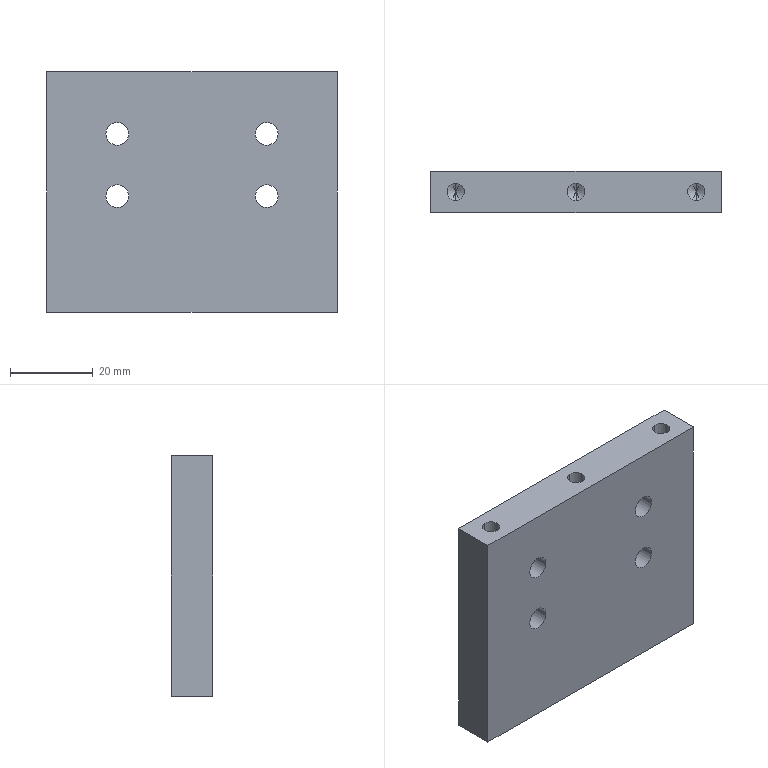Component | SolidWorks | LD101-02--Q1000-Q16-1.SLDQ1SM-1_LD101-02--Q1109-1-2 | 1 solid | 50 faces | box 70 x 10 x 58 mm | volume 37509 mm3 | cylinder 28 | cone 12 | plane 10 | commonest cylinder face diameters 4.2 x12 9 x8 5.5 x8 | material AL6061
build123d program:
from build123d import *

# Parameters (mm, degrees)
SKETCH1_W                                          = 70
SKETCH1_H                                          = 58
BOSS_EXTRUDE1_DEPTH                                = 5
M5_TAPPED_HOLE1_AT_2_COUNT                         = 2
M5_TAPPED_HOLE1_AT_2_PITCH                         = 58
M5_TAPPED_HOLE1_AT_3_COUNT                         = 2
M5_TAPPED_HOLE1_AT_3_PITCH                         = 29
HOLE_SIZE_FOR_HEX_SOCKET_HEAD_CAP_SCRE_D           = 5.5
HOLE_SIZE_FOR_HEX_SOCKET_HEAD_CAP_SCRE_CBORE_D     = 9
HOLE_SIZE_FOR_HEX_SOCKET_HEAD_CAP_SCRE_CBORE_DEPTH = 5.7


with BuildPart() as part:
    # Sketch1 → Boss-Extrude1 (new, symmetric)
    with BuildSketch(Plane.XY):
        Rectangle(SKETCH1_W, SKETCH1_H)
    extrude(amount=BOSS_EXTRUDE1_DEPTH, both=True)

    # Sketch2 → M5 Tapped Hole1 (revolve, cut)
    with BuildSketch(Plane(origin=(-29, 29, 0), x_dir=(0, 0, 1), z_dir=(1, 0, 0))):
        Polygon((0, 0), (0, 15.662), (2.1, 14.4), (2.1, 0), align=None)
    m5_tapped_hole1 = revolve(axis=Axis((-29, 35.35, 0), (0, -1, 0)), mode=Mode.SUBTRACT)

    # M5 Tapped Hole1 at 2: M5 Tapped Hole1 ×2
    with Locations(*[(i * M5_TAPPED_HOLE1_AT_2_PITCH, 0, 0) for i in range(1, M5_TAPPED_HOLE1_AT_2_COUNT)]):
        add(m5_tapped_hole1, mode=Mode.SUBTRACT)

    # M5 Tapped Hole1 at 3: M5 Tapped Hole1 ×2
    with Locations(*[(i * M5_TAPPED_HOLE1_AT_3_PITCH, 0, 0) for i in range(1, M5_TAPPED_HOLE1_AT_3_COUNT)]):
        add(m5_tapped_hole1, mode=Mode.SUBTRACT)

    # Mirror1: M5 Tapped Hole1 across plane
    add(m5_tapped_hole1.mirror(Plane.ZX), mode=Mode.SUBTRACT)

    # Mirror1 copy 1 sketch → Mirror1 copy 1 (revolve, cut)
    with BuildSketch(Plane(origin=(29, -29, 0), x_dir=(0, 0, 1), z_dir=(1, 0, 0))):
        Polygon((0, 0), (0, -15.662), (2.1, -14.4), (2.1, 0), align=None)
    revolve(axis=Axis((29, -35.35, 0), (0, -1, 0)), mode=Mode.SUBTRACT)

    # Mirror1 copy 2 sketch → Mirror1 copy 2 (revolve, cut)
    with BuildSketch(Plane(origin=(0, -29, 0), x_dir=(0, 0, 1), z_dir=(1, 0, 0))):
        Polygon((0, 0), (0, -15.662), (2.1, -14.4), (2.1, 0), align=None)
    revolve(axis=Axis((0, -35.35, 0), (0, -1, 0)), mode=Mode.SUBTRACT)

    # Hole Size _for_ Hex Socket Head Cap Scre (through all)
    with Locations(Plane(origin=(0, 0, -5), x_dir=(-1, 0, 0), z_dir=(0, 0, -1))):
        with Locations((-18, 1), (18, 1), (-18, -14), (18, -14)):
            CounterBoreHole(HOLE_SIZE_FOR_HEX_SOCKET_HEAD_CAP_SCRE_D / 2, HOLE_SIZE_FOR_HEX_SOCKET_HEAD_CAP_SCRE_CBORE_D / 2, HOLE_SIZE_FOR_HEX_SOCKET_HEAD_CAP_SCRE_CBORE_DEPTH)


solid = part.part

# Placed as in the assembly
solid = solid.moved(Location((-753.29, -134.897, -41.743), (90, 0, -180)))